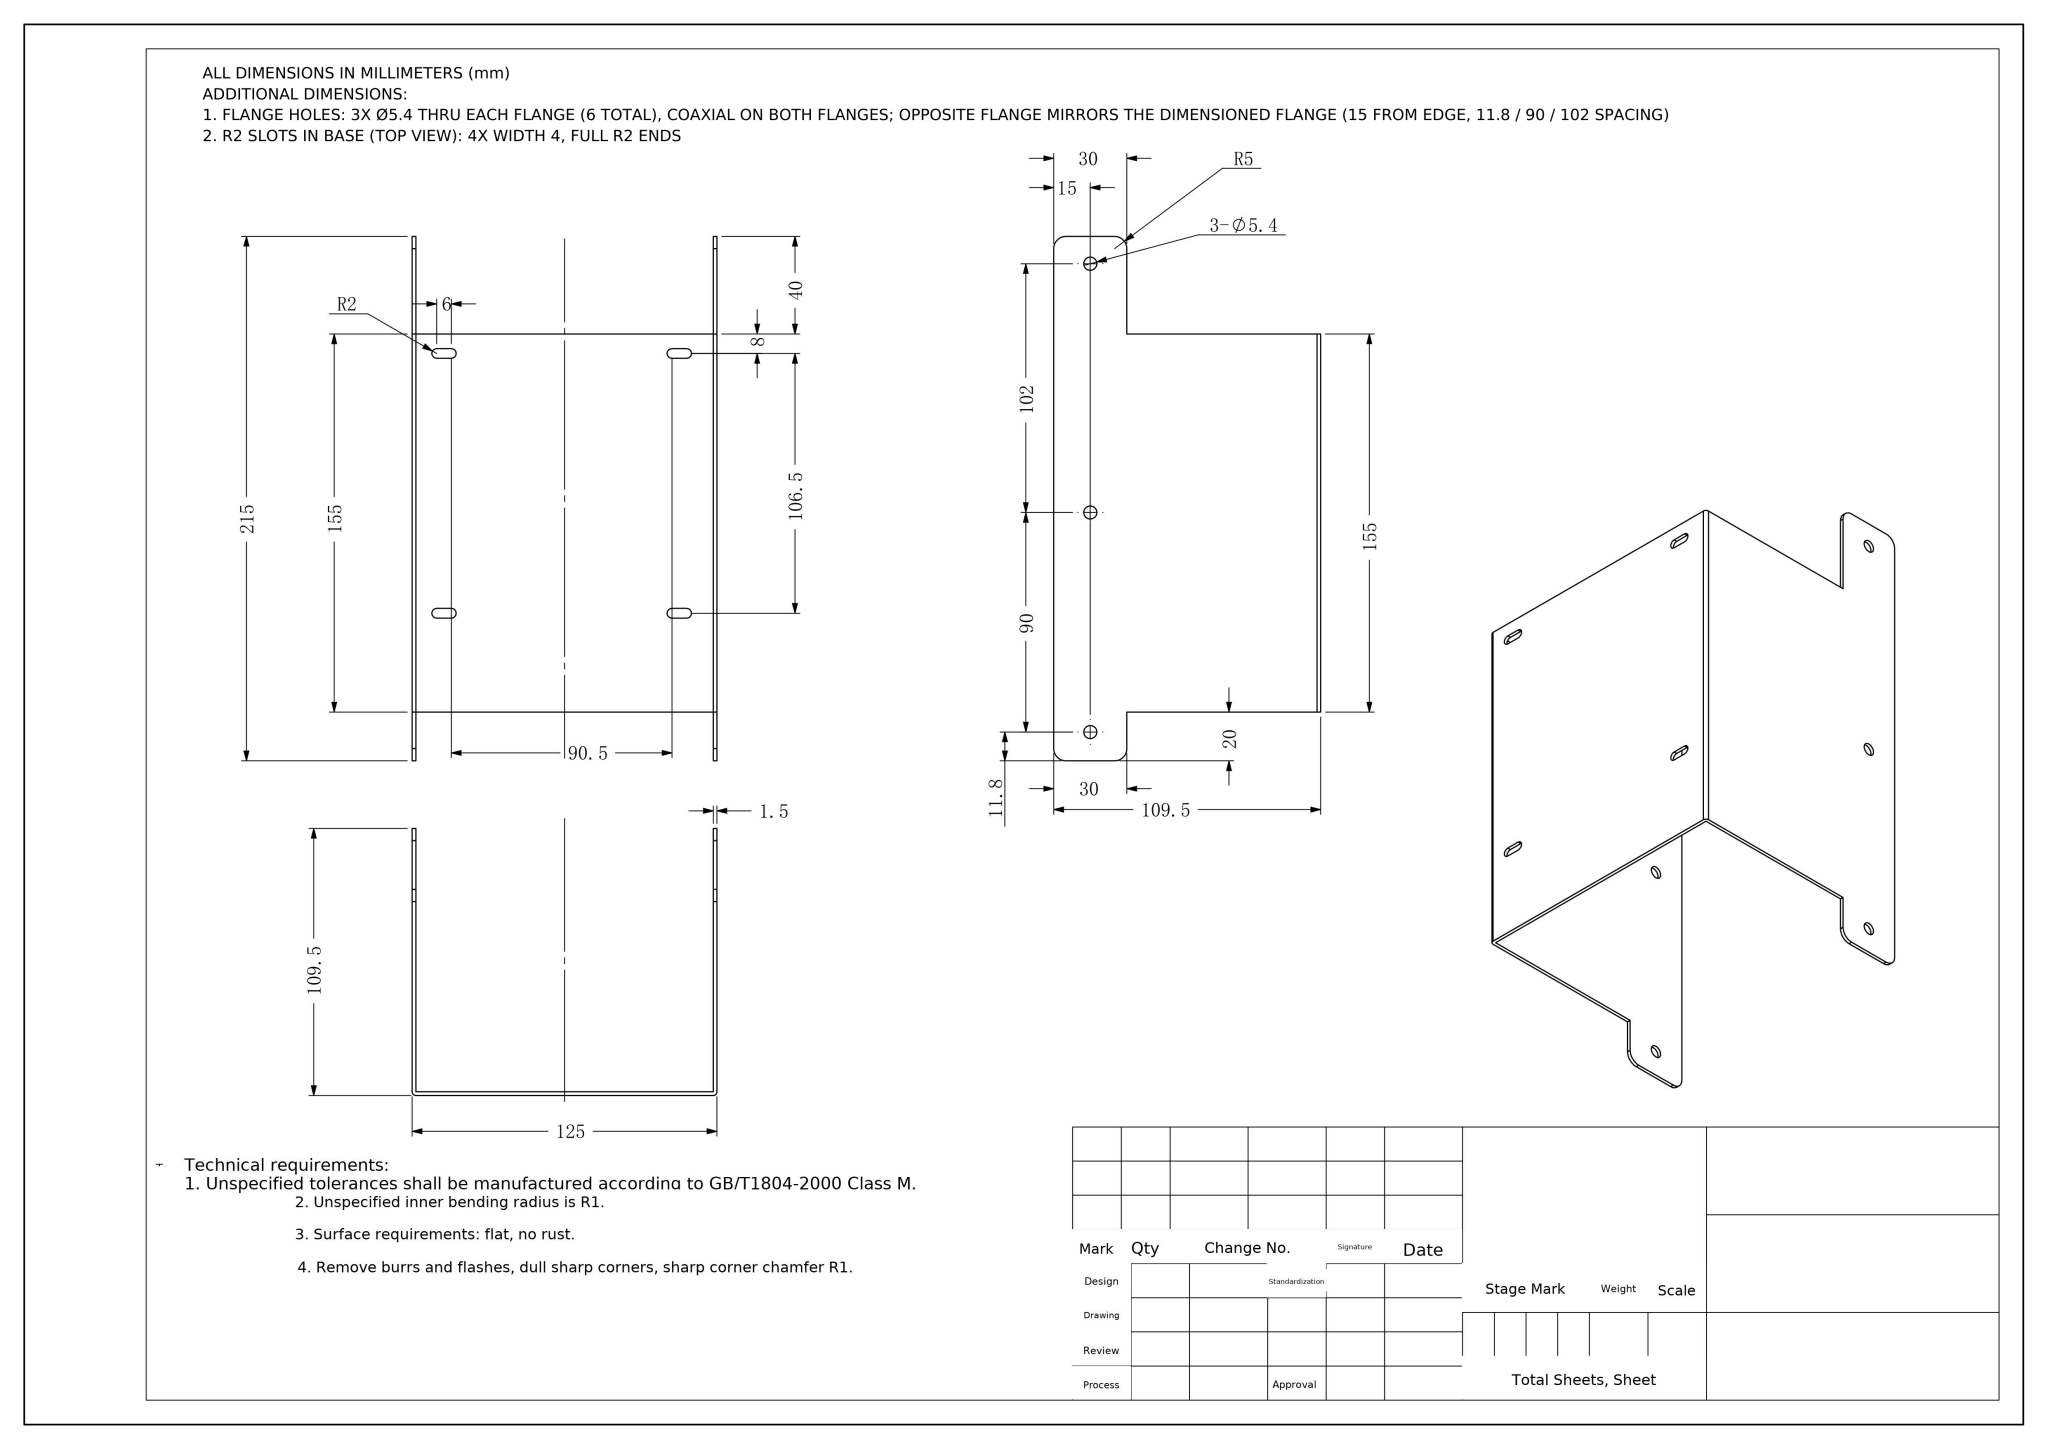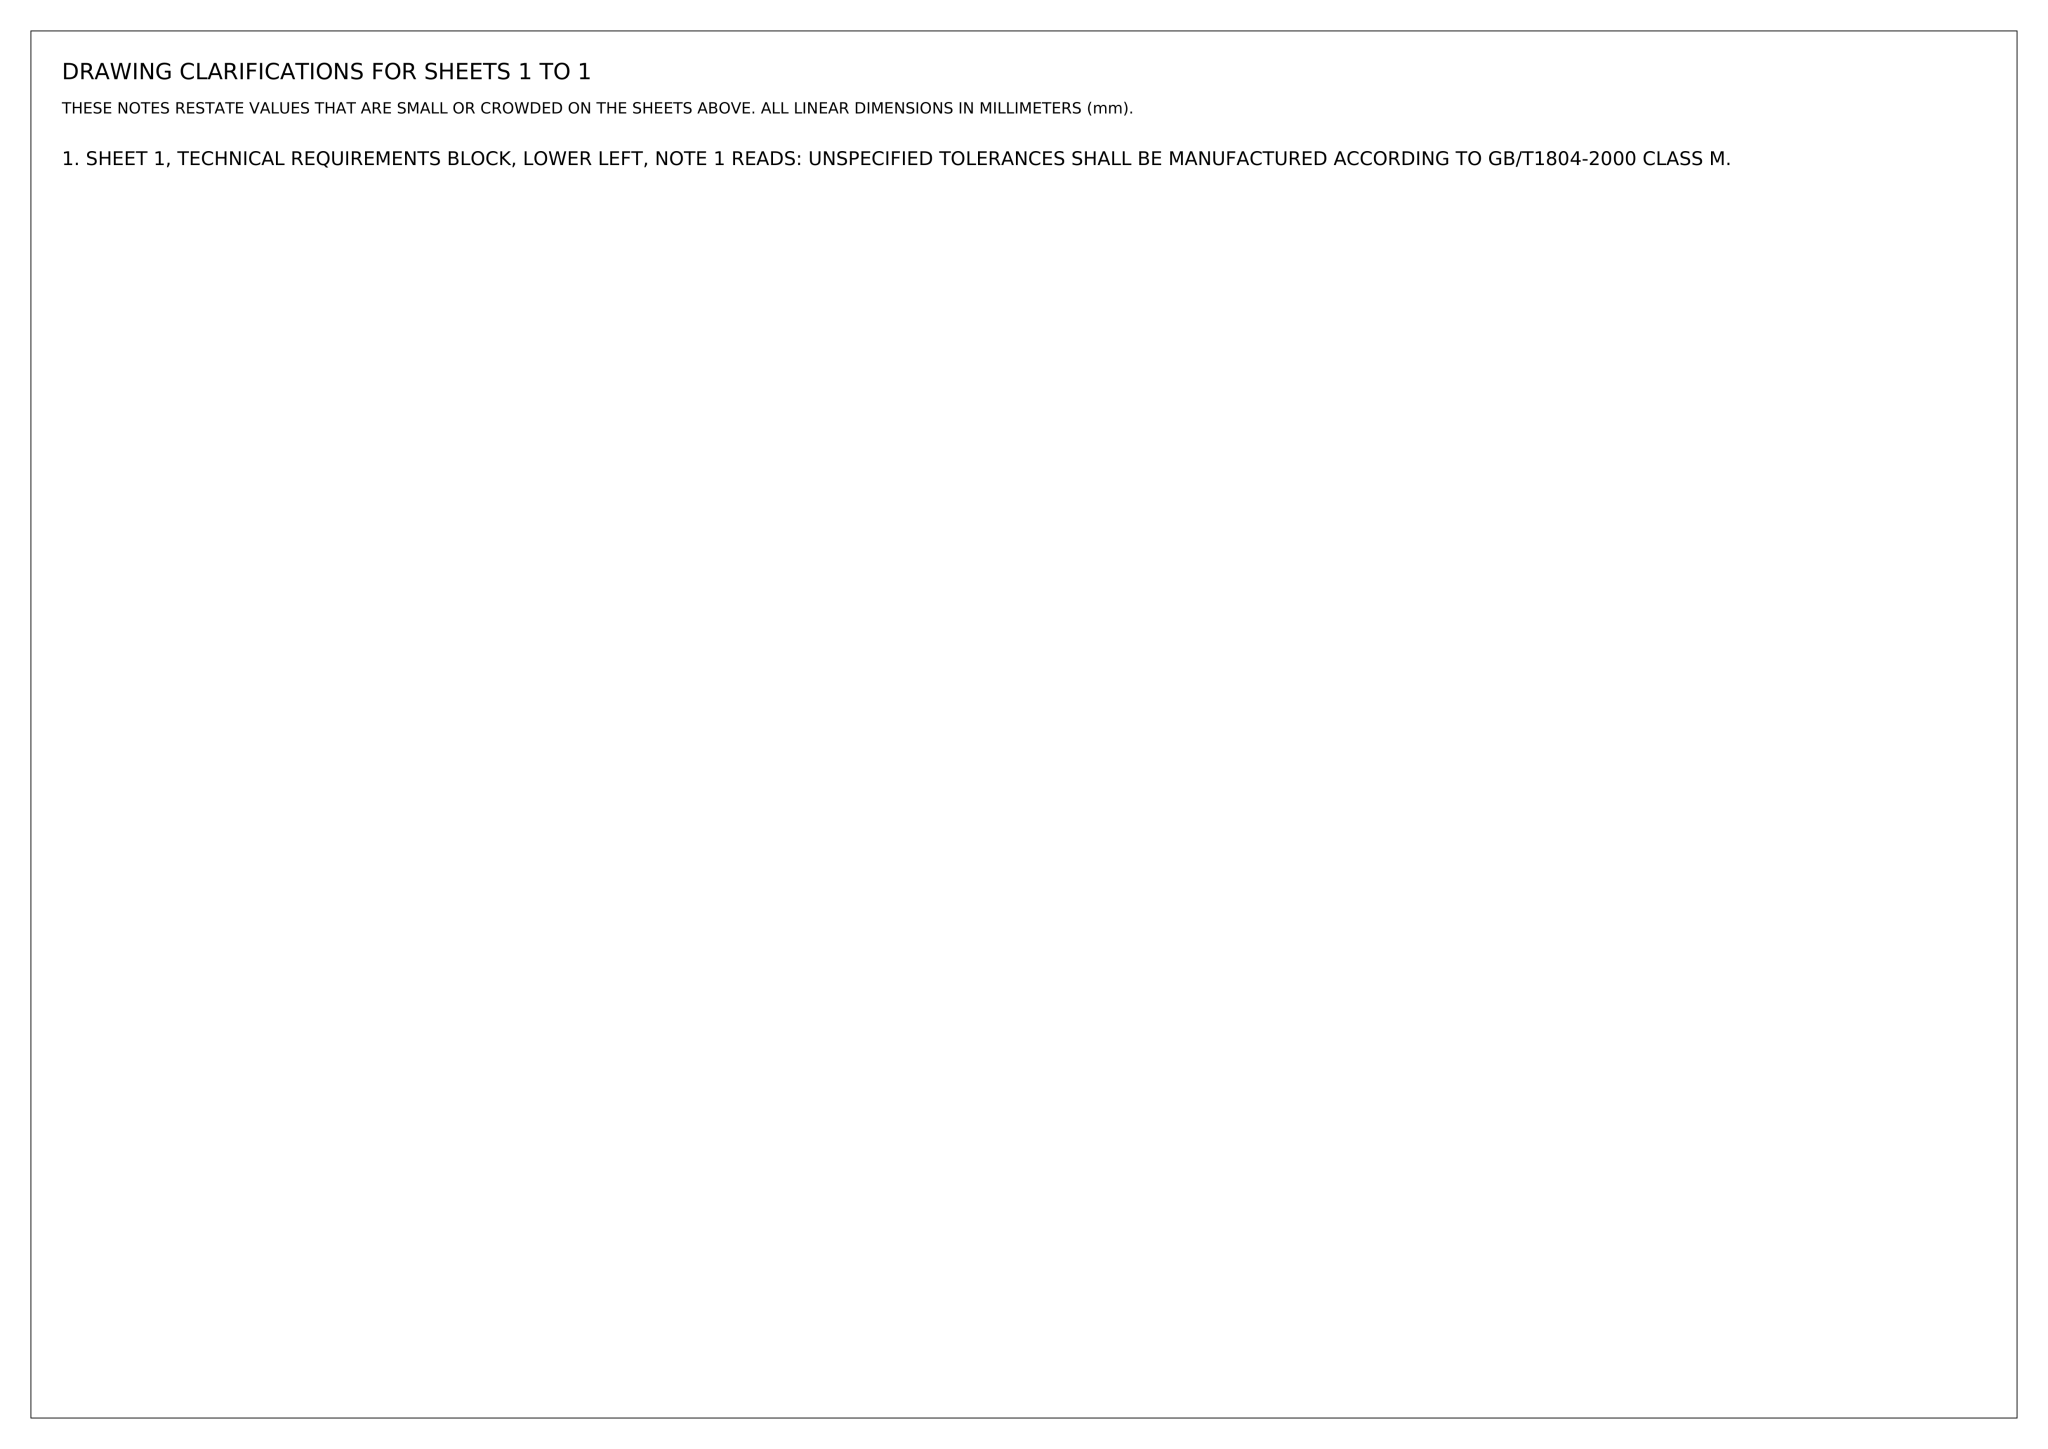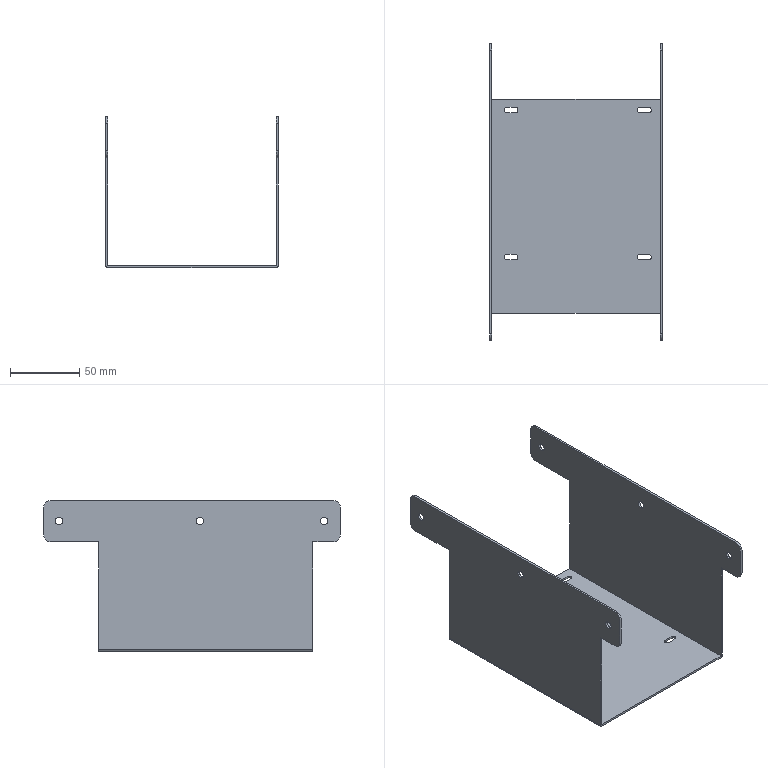Part | NX | mm | 1 solid | 62 faces | box 125 x 215 x 109.5 mm | volume 84043 mm3 | cylinder 36 | plane 26 | commonest cylinder face diameters 5.4 x12 4 x12 10 x8 3.004 x2 0.004 x2